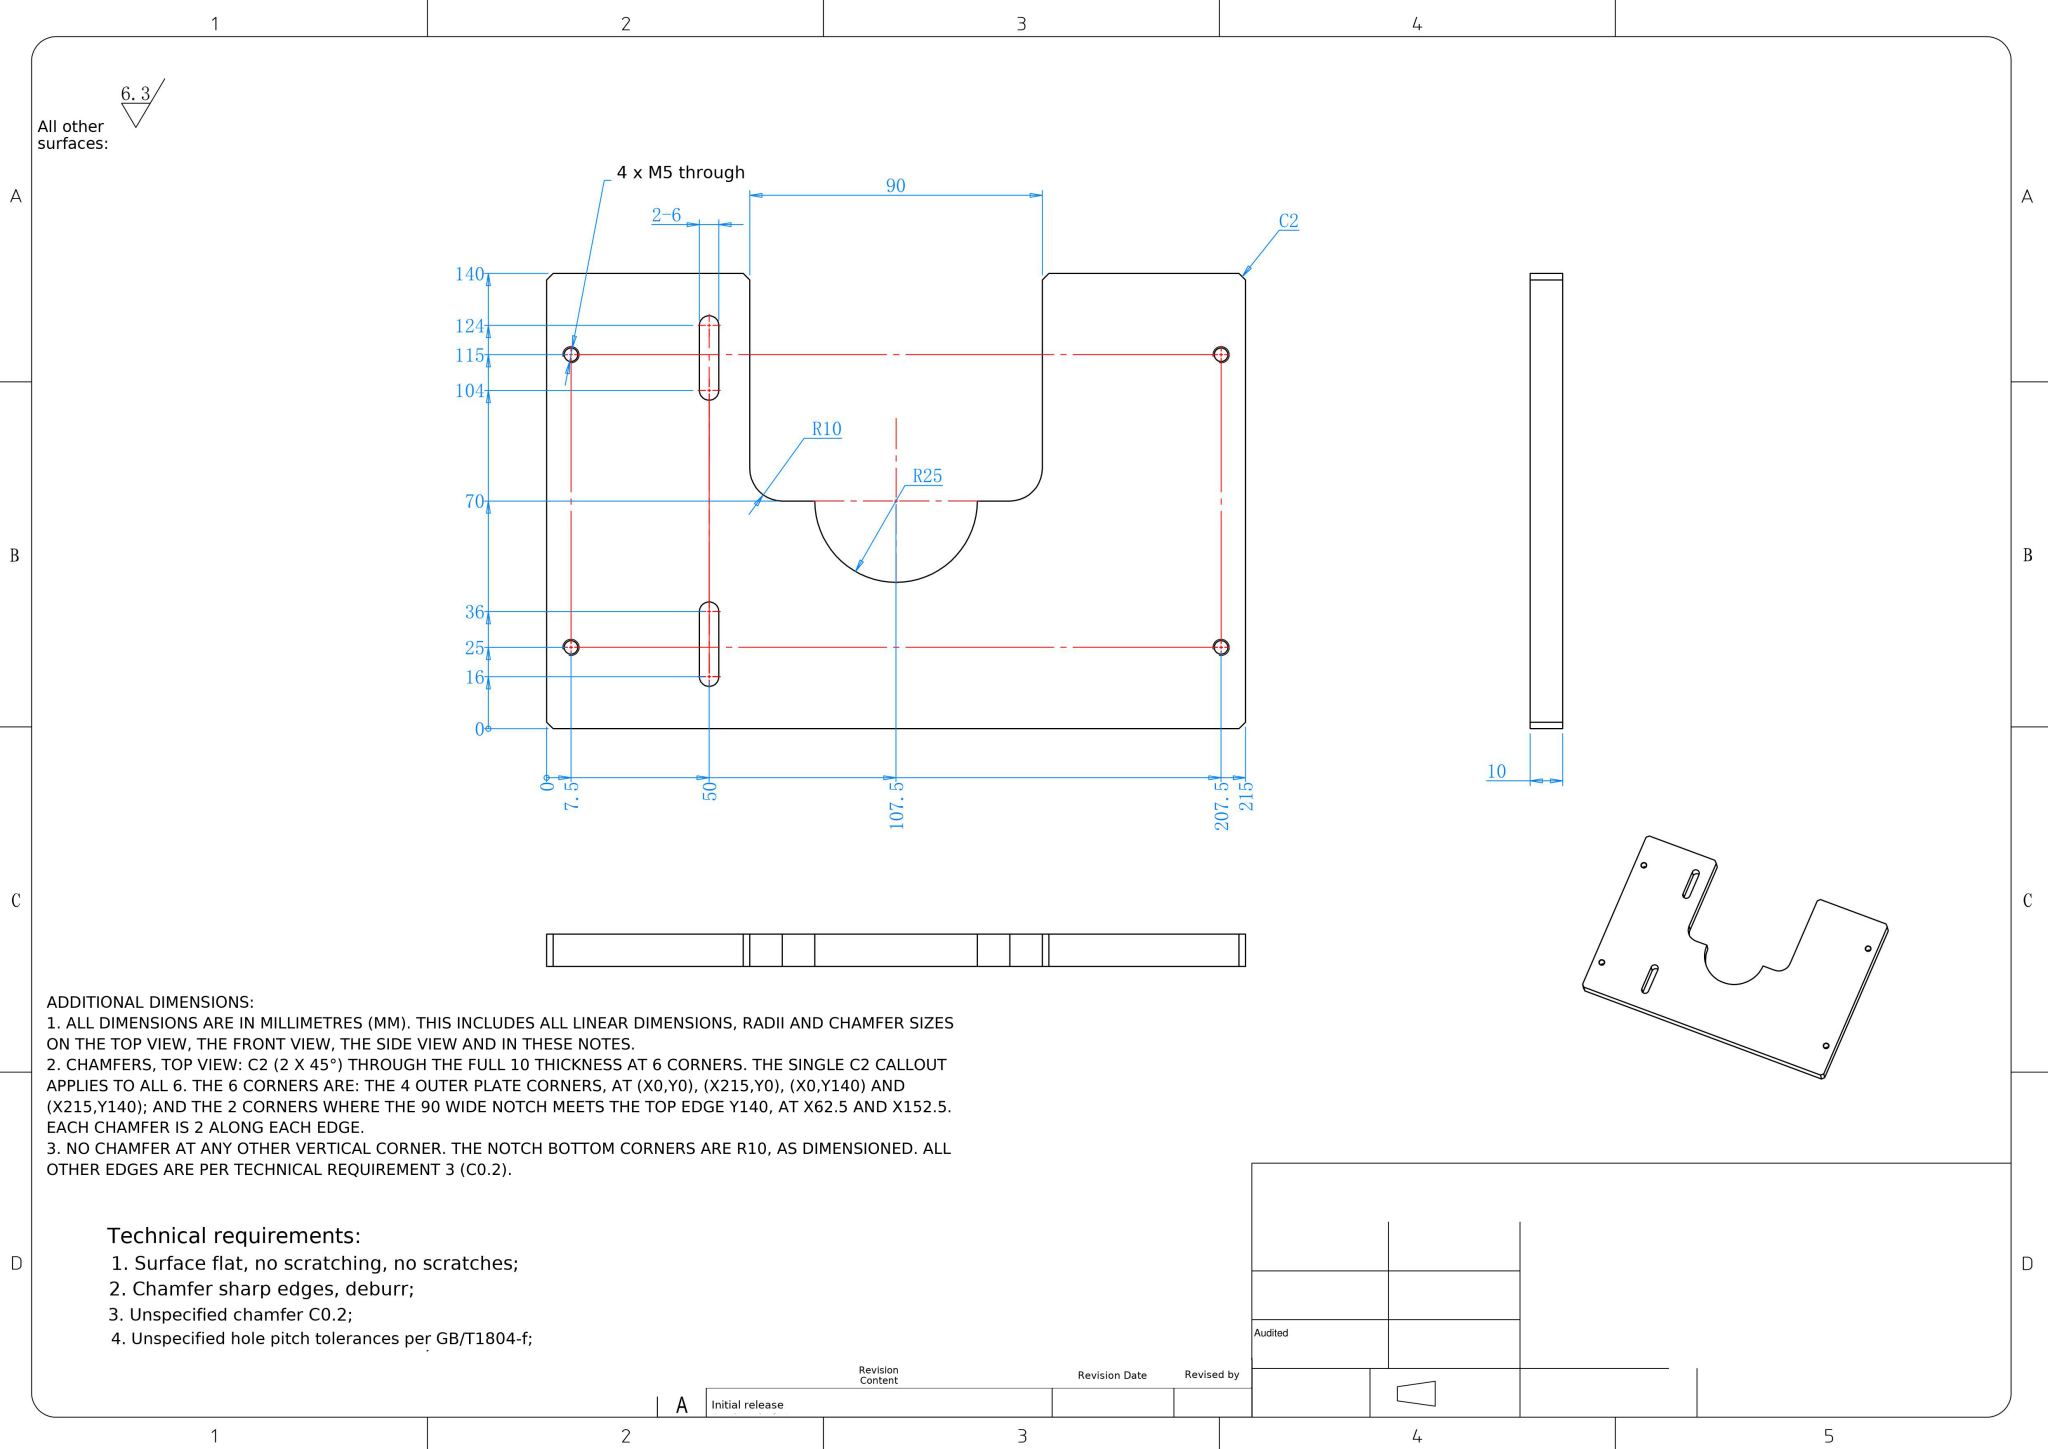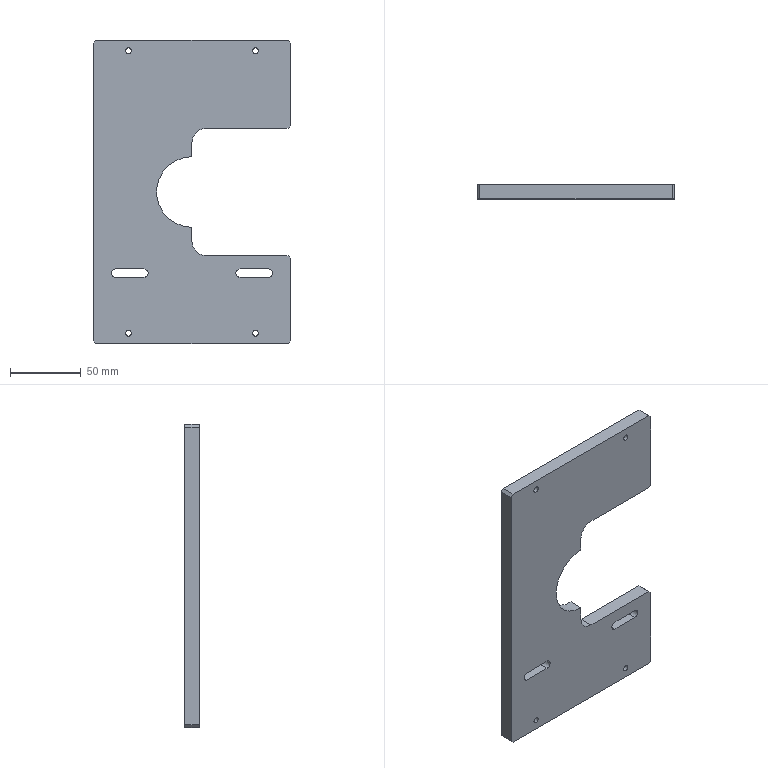Part | NX | mm | 1 solid | 36 faces | box 140 x 10 x 215 mm | volume 224972 mm3 | plane 21 | cylinder 15 | commonest cylinder face diameters 4.2 x8 6 x4 20 x2 50 x1